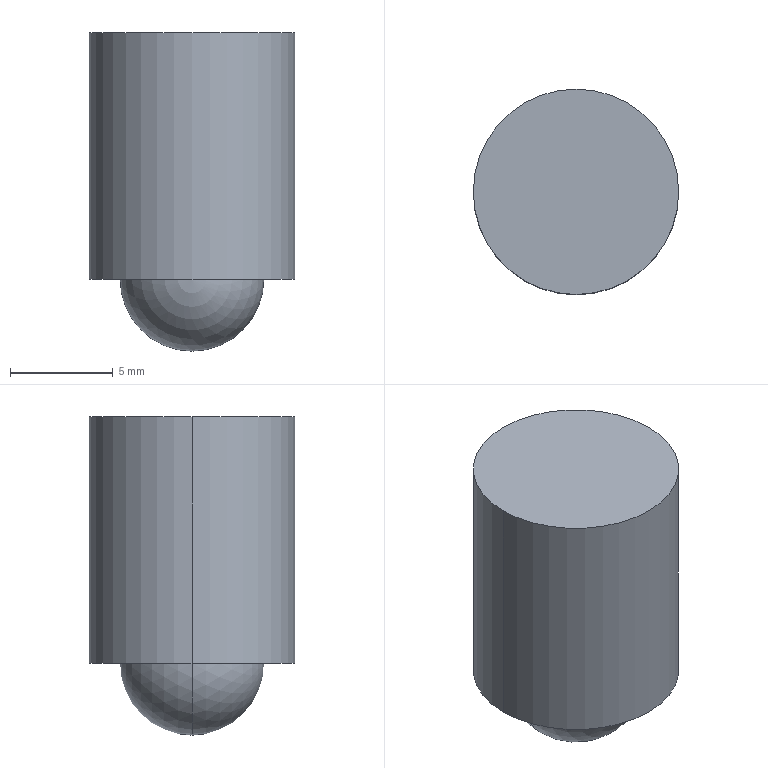Component | SolidWorks | BallPlungerM10X12-1 | 1 solid | 6 faces | box 10 x 10 x 15.5 mm | volume 1032 mm3 | sphere 2 | cylinder 2 | plane 2 | commonest cylinder face diameters 10 x2
build123d program:
from build123d import *

# Parameters (mm, degrees)
SKETCH1_W = 12
SKETCH1_H = 5


with BuildPart() as part:
    # Sketch1 → Revolve1 (revolve)
    with BuildSketch(Plane(origin=(0, 0, 0), x_dir=(0, 0, -1), z_dir=(1, 0, 0)), mode=Mode.PRIVATE) as revolve1_sk:
        with Locations((6, 2.5)):
            Rectangle(SKETCH1_W, SKETCH1_H)
    revolve(revolve1_sk.sketch.rotate(Axis((0, 0, 50.996), (0, 0, -1)), 90), axis=Axis((0, 0, 50.996), (0, 0, -1)))

    # Sketch2 → Revolve2 (revolve)
    with BuildSketch(Plane(origin=(0, 0, 0), x_dir=(1, 0, 0), z_dir=(0, 1, 0)), mode=Mode.PRIVATE) as revolve2_sk:
        with BuildLine():
            Line((-3.5, 12), (0, 12))
            Line((0, 12), (0, 15.5))
            ThreePointArc((0, 15.5), (-2.475, 14.475), (-3.5, 12))
        make_face()
    revolve(revolve2_sk.sketch.rotate(Axis((0, 0, 0), (0, 0, -1)), 180), axis=Axis((0, 0, 0), (0, 0, -1)))


solid = part.part

# Placed as in the assembly
solid = solid.moved(Location((7.266, 69.299, 68), (0, 0, 0)))
STEP:
#1=COLOUR_RGB('',0.7922,0.8196,0.9333);
#2=FILL_AREA_STYLE_COLOUR('',#1);
#3=FILL_AREA_STYLE('',(#2));
#4=SURFACE_STYLE_FILL_AREA(#3);
#5=SURFACE_SIDE_STYLE('',(#4));
#6=SURFACE_STYLE_USAGE(.BOTH.,#5);
#7=PRESENTATION_STYLE_ASSIGNMENT((#6));
#8=CARTESIAN_POINT('',(0.2861,2.728,2.067));
#9=VERTEX_POINT('',#8);
#10=CARTESIAN_POINT('',(0.4239,2.728,2.205));
#11=VERTEX_POINT('',#10);
#12=CARTESIAN_POINT('',(0.2861,2.728,2.205));
#13=DIRECTION('',(0.,-1.,0.));
#14=DIRECTION('',(0.,0.,-1.));
#15=AXIS2_PLACEMENT_3D('',#12,#13,#14);
#16=CIRCLE('',#15,0.1378);
#17=EDGE_CURVE('',#9,#11,#16,.T.);
#18=ORIENTED_EDGE('',*,*,#17,.F.);
#19=CARTESIAN_POINT('',(0.1483,2.728,2.205));
#20=VERTEX_POINT('',#19);
#21=CARTESIAN_POINT('',(0.2861,2.728,2.205));
#22=DIRECTION('',(0.,1.,0.));
#23=DIRECTION('',(-1.,0.,0.));
#24=AXIS2_PLACEMENT_3D('',#21,#22,#23);
#25=CIRCLE('',#24,0.1378);
#26=EDGE_CURVE('',#9,#20,#25,.T.);
#27=ORIENTED_EDGE('',*,*,#26,.T.);
#28=CARTESIAN_POINT('',(0.2861,2.728,2.205));
#29=DIRECTION('',(0.,0.,-1.));
#30=DIRECTION('',(1.,0.,0.));
#31=AXIS2_PLACEMENT_3D('',#28,#29,#30);
#32=CIRCLE('',#31,0.1378);
#33=EDGE_CURVE('',#20,#11,#32,.T.);
#34=ORIENTED_EDGE('',*,*,#33,.T.);
#35=EDGE_LOOP('',(#18,#27,#34));
#36=FACE_OUTER_BOUND('',#35,.T.);
#37=CARTESIAN_POINT('',(0.2861,2.728,2.205));
#38=DIRECTION('',(0.,1.,0.));
#39=DIRECTION('',(1.,0.,0.));
#40=AXIS2_PLACEMENT_3D('',#37,#38,#39);
#41=SPHERICAL_SURFACE('',#40,0.1378);
#42=ADVANCED_FACE('',(#36),#41,.T.);
#43=CARTESIAN_POINT('',(0.4829,2.728,2.205));
#44=VERTEX_POINT('',#43);
#45=CARTESIAN_POINT('',(0.08922,2.728,2.205));
#46=VERTEX_POINT('',#45);
#47=CARTESIAN_POINT('',(0.2861,2.728,2.205));
#48=DIRECTION('',(0.,0.,1.));
#49=DIRECTION('',(1.,0.,0.));
#50=AXIS2_PLACEMENT_3D('',#47,#48,#49);
#51=CIRCLE('',#50,0.1969);
#52=EDGE_CURVE('',#44,#46,#51,.T.);
#53=ORIENTED_EDGE('',*,*,#52,.T.);
#54=CARTESIAN_POINT('',(0.08922,2.728,2.677));
#55=VERTEX_POINT('',#54);
#56=CARTESIAN_POINT('',(0.08922,2.728,4.685));
#57=DIRECTION('',(0.,0.,1.));
#58=VECTOR('',#57,39.37);
#59=LINE('',#56,#58);
#60=EDGE_CURVE('',#46,#55,#59,.T.);
#61=ORIENTED_EDGE('',*,*,#60,.T.);
#62=CARTESIAN_POINT('',(0.4829,2.728,2.677));
#63=VERTEX_POINT('',#62);
#64=CARTESIAN_POINT('',(0.2861,2.728,2.677));
#65=DIRECTION('',(0.,0.,1.));
#66=DIRECTION('',(1.,0.,0.));
#67=AXIS2_PLACEMENT_3D('',#64,#65,#66);
#68=CIRCLE('',#67,0.1969);
#69=EDGE_CURVE('',#63,#55,#68,.T.);
#70=ORIENTED_EDGE('',*,*,#69,.F.);
#71=CARTESIAN_POINT('',(0.4829,2.728,4.685));
#72=DIRECTION('',(0.,0.,1.));
#73=VECTOR('',#72,39.37);
#74=LINE('',#71,#73);
#75=EDGE_CURVE('',#44,#63,#74,.T.);
#76=ORIENTED_EDGE('',*,*,#75,.F.);
#77=EDGE_LOOP('',(#53,#61,#70,#76));
#78=FACE_OUTER_BOUND('',#77,.T.);
#79=CARTESIAN_POINT('',(0.2861,2.728,4.685));
#80=DIRECTION('',(0.,0.,1.));
#81=DIRECTION('',(1.,0.,0.));
#82=AXIS2_PLACEMENT_3D('',#79,#80,#81);
#83=CYLINDRICAL_SURFACE('',#82,0.1969);
#84=ADVANCED_FACE('',(#78),#83,.T.);
#85=ORIENTED_EDGE('',*,*,#52,.F.);
#86=CARTESIAN_POINT('',(0.2861,2.728,2.205));
#87=DIRECTION('',(0.,0.,1.));
#88=DIRECTION('',(1.,0.,0.));
#89=AXIS2_PLACEMENT_3D('',#86,#87,#88);
#90=CIRCLE('',#89,0.1969);
#91=EDGE_CURVE('',#46,#44,#90,.T.);
#92=ORIENTED_EDGE('',*,*,#91,.F.);
#93=EDGE_LOOP('',(#85,#92));
#94=FACE_OUTER_BOUND('',#93,.T.);
#95=CARTESIAN_POINT('',(0.2861,2.728,2.205));
#96=DIRECTION('',(0.,0.,-1.));
#97=DIRECTION('',(1.,0.,0.));
#98=AXIS2_PLACEMENT_3D('',#95,#96,#97);
#99=CIRCLE('',#98,0.1378);
#100=EDGE_CURVE('',#11,#20,#99,.T.);
#101=ORIENTED_EDGE('',*,*,#100,.F.);
#102=ORIENTED_EDGE('',*,*,#33,.F.);
#103=EDGE_LOOP('',(#101,#102));
#104=FACE_BOUND('',#103,.T.);
#105=CARTESIAN_POINT('',(0.2861,2.925,2.205));
#106=DIRECTION('',(0.,0.,1.));
#107=DIRECTION('',(1.,0.,0.));
#108=AXIS2_PLACEMENT_3D('',#105,#106,#107);
#109=PLANE('',#108);
#110=ADVANCED_FACE('',(#94,#104),#109,.F.);
#111=ORIENTED_EDGE('',*,*,#69,.T.);
#112=CARTESIAN_POINT('',(0.2861,2.728,2.677));
#113=DIRECTION('',(0.,0.,1.));
#114=DIRECTION('',(1.,0.,0.));
#115=AXIS2_PLACEMENT_3D('',#112,#113,#114);
#116=CIRCLE('',#115,0.1969);
#117=EDGE_CURVE('',#55,#63,#116,.T.);
#118=ORIENTED_EDGE('',*,*,#117,.T.);
#119=EDGE_LOOP('',(#111,#118));
#120=FACE_OUTER_BOUND('',#119,.T.);
#121=CARTESIAN_POINT('',(0.2861,2.728,2.677));
#122=DIRECTION('',(0.,0.,-1.));
#123=DIRECTION('',(-1.,0.,0.));
#124=AXIS2_PLACEMENT_3D('',#121,#122,#123);
#125=PLANE('',#124);
#126=ADVANCED_FACE('',(#120),#125,.F.);
#127=ORIENTED_EDGE('',*,*,#60,.F.);
#128=ORIENTED_EDGE('',*,*,#91,.T.);
#129=ORIENTED_EDGE('',*,*,#75,.T.);
#130=ORIENTED_EDGE('',*,*,#117,.F.);
#131=EDGE_LOOP('',(#127,#128,#129,#130));
#132=FACE_OUTER_BOUND('',#131,.T.);
#133=CARTESIAN_POINT('',(0.2861,2.728,4.685));
#134=DIRECTION('',(0.,0.,1.));
#135=DIRECTION('',(1.,0.,0.));
#136=AXIS2_PLACEMENT_3D('',#133,#134,#135);
#137=CYLINDRICAL_SURFACE('',#136,0.1969);
#138=ADVANCED_FACE('',(#132),#137,.T.);
#139=ORIENTED_EDGE('',*,*,#26,.F.);
#140=ORIENTED_EDGE('',*,*,#17,.T.);
#141=ORIENTED_EDGE('',*,*,#100,.T.);
#142=EDGE_LOOP('',(#139,#140,#141));
#143=FACE_OUTER_BOUND('',#142,.T.);
#144=CARTESIAN_POINT('',(0.2861,2.728,2.205));
#145=DIRECTION('',(0.,1.,0.));
#146=DIRECTION('',(1.,0.,0.));
#147=AXIS2_PLACEMENT_3D('',#144,#145,#146);
#148=SPHERICAL_SURFACE('',#147,0.1378);
#149=ADVANCED_FACE('',(#143),#148,.T.);
#150=CLOSED_SHELL('',(#42,#84,#110,#126,#138,#149));
#151=MANIFOLD_SOLID_BREP('',#150);
#152=STYLED_ITEM('',(#7),#151);
#153=PRESENTATION_LAYER_ASSIGNMENT('','',(#152));
#154=(LENGTH_UNIT()NAMED_UNIT(*)SI_UNIT($,.METRE.));
#155=LENGTH_MEASURE_WITH_UNIT(LENGTH_MEASURE(0.0254),#154);
#156=DIMENSIONAL_EXPONENTS(1.,0.,0.,0.,0.,0.,0.);
#157=(CONVERSION_BASED_UNIT('',#155)LENGTH_UNIT()NAMED_UNIT(#156));
#158=UNCERTAINTY_MEASURE_WITH_UNIT(LENGTH_MEASURE(0.00001),#157,'','');
#159=(NAMED_UNIT(*)PLANE_ANGLE_UNIT()SI_UNIT($,.RADIAN.));
#160=(NAMED_UNIT(*)SI_UNIT($,.STERADIAN.)SOLID_ANGLE_UNIT());
#161=(GEOMETRIC_REPRESENTATION_CONTEXT(3)GLOBAL_UNCERTAINTY_ASSIGNED_CONTEXT((#158))GLOBAL_UNIT_ASSIGNED_CONTEXT((#157,#159,#160))REPRESENTATION_CONTEXT('',''));
#162=MECHANICAL_DESIGN_GEOMETRIC_PRESENTATION_REPRESENTATION('',(#152),#161);
#163=CARTESIAN_POINT('',(0.,0.,0.));
#164=DIRECTION('',(0.,0.,1.));
#165=DIRECTION('',(1.,0.,0.));
#166=AXIS2_PLACEMENT_3D('',#163,#164,#165);
#167=(LENGTH_UNIT()NAMED_UNIT(*)SI_UNIT($,.METRE.));
#168=LENGTH_MEASURE_WITH_UNIT(LENGTH_MEASURE(0.0254),#167);
#169=DIMENSIONAL_EXPONENTS(1.,0.,0.,0.,0.,0.,0.);
#170=(CONVERSION_BASED_UNIT('',#168)LENGTH_UNIT()NAMED_UNIT(#169));
#171=UNCERTAINTY_MEASURE_WITH_UNIT(LENGTH_MEASURE(0.00001),#170,'','');
#172=(NAMED_UNIT(*)PLANE_ANGLE_UNIT()SI_UNIT($,.RADIAN.));
#173=(NAMED_UNIT(*)SI_UNIT($,.STERADIAN.)SOLID_ANGLE_UNIT());
#174=(GEOMETRIC_REPRESENTATION_CONTEXT(3)GLOBAL_UNCERTAINTY_ASSIGNED_CONTEXT((#171))GLOBAL_UNIT_ASSIGNED_CONTEXT((#170,#172,#173))REPRESENTATION_CONTEXT('',''));
#175=ADVANCED_BREP_SHAPE_REPRESENTATION('',(#151,#166),#174);